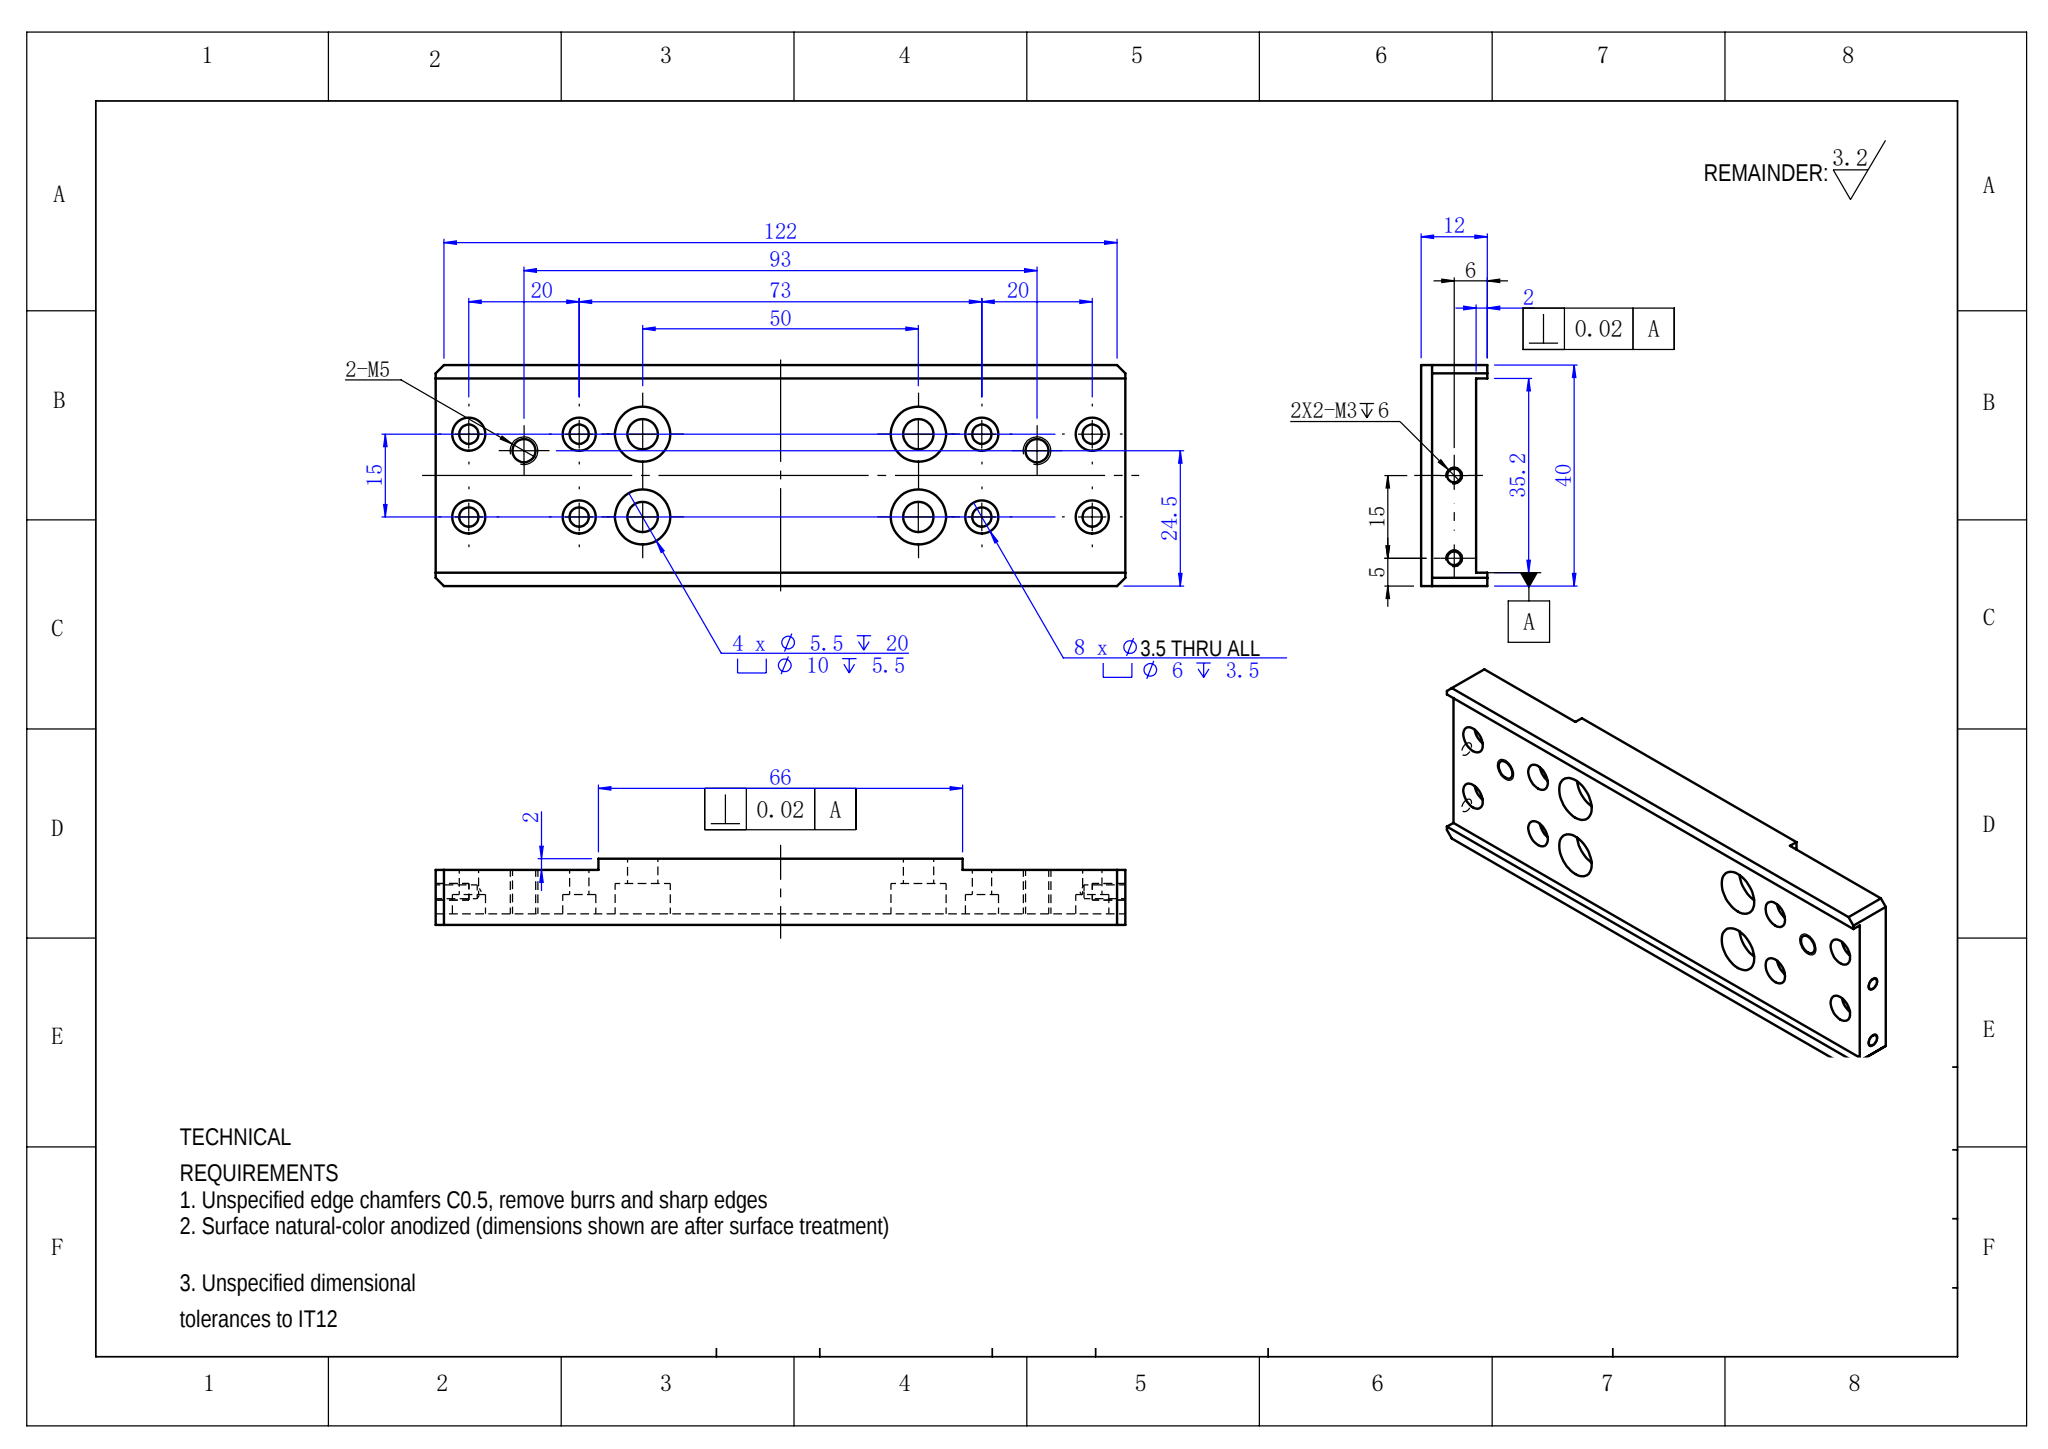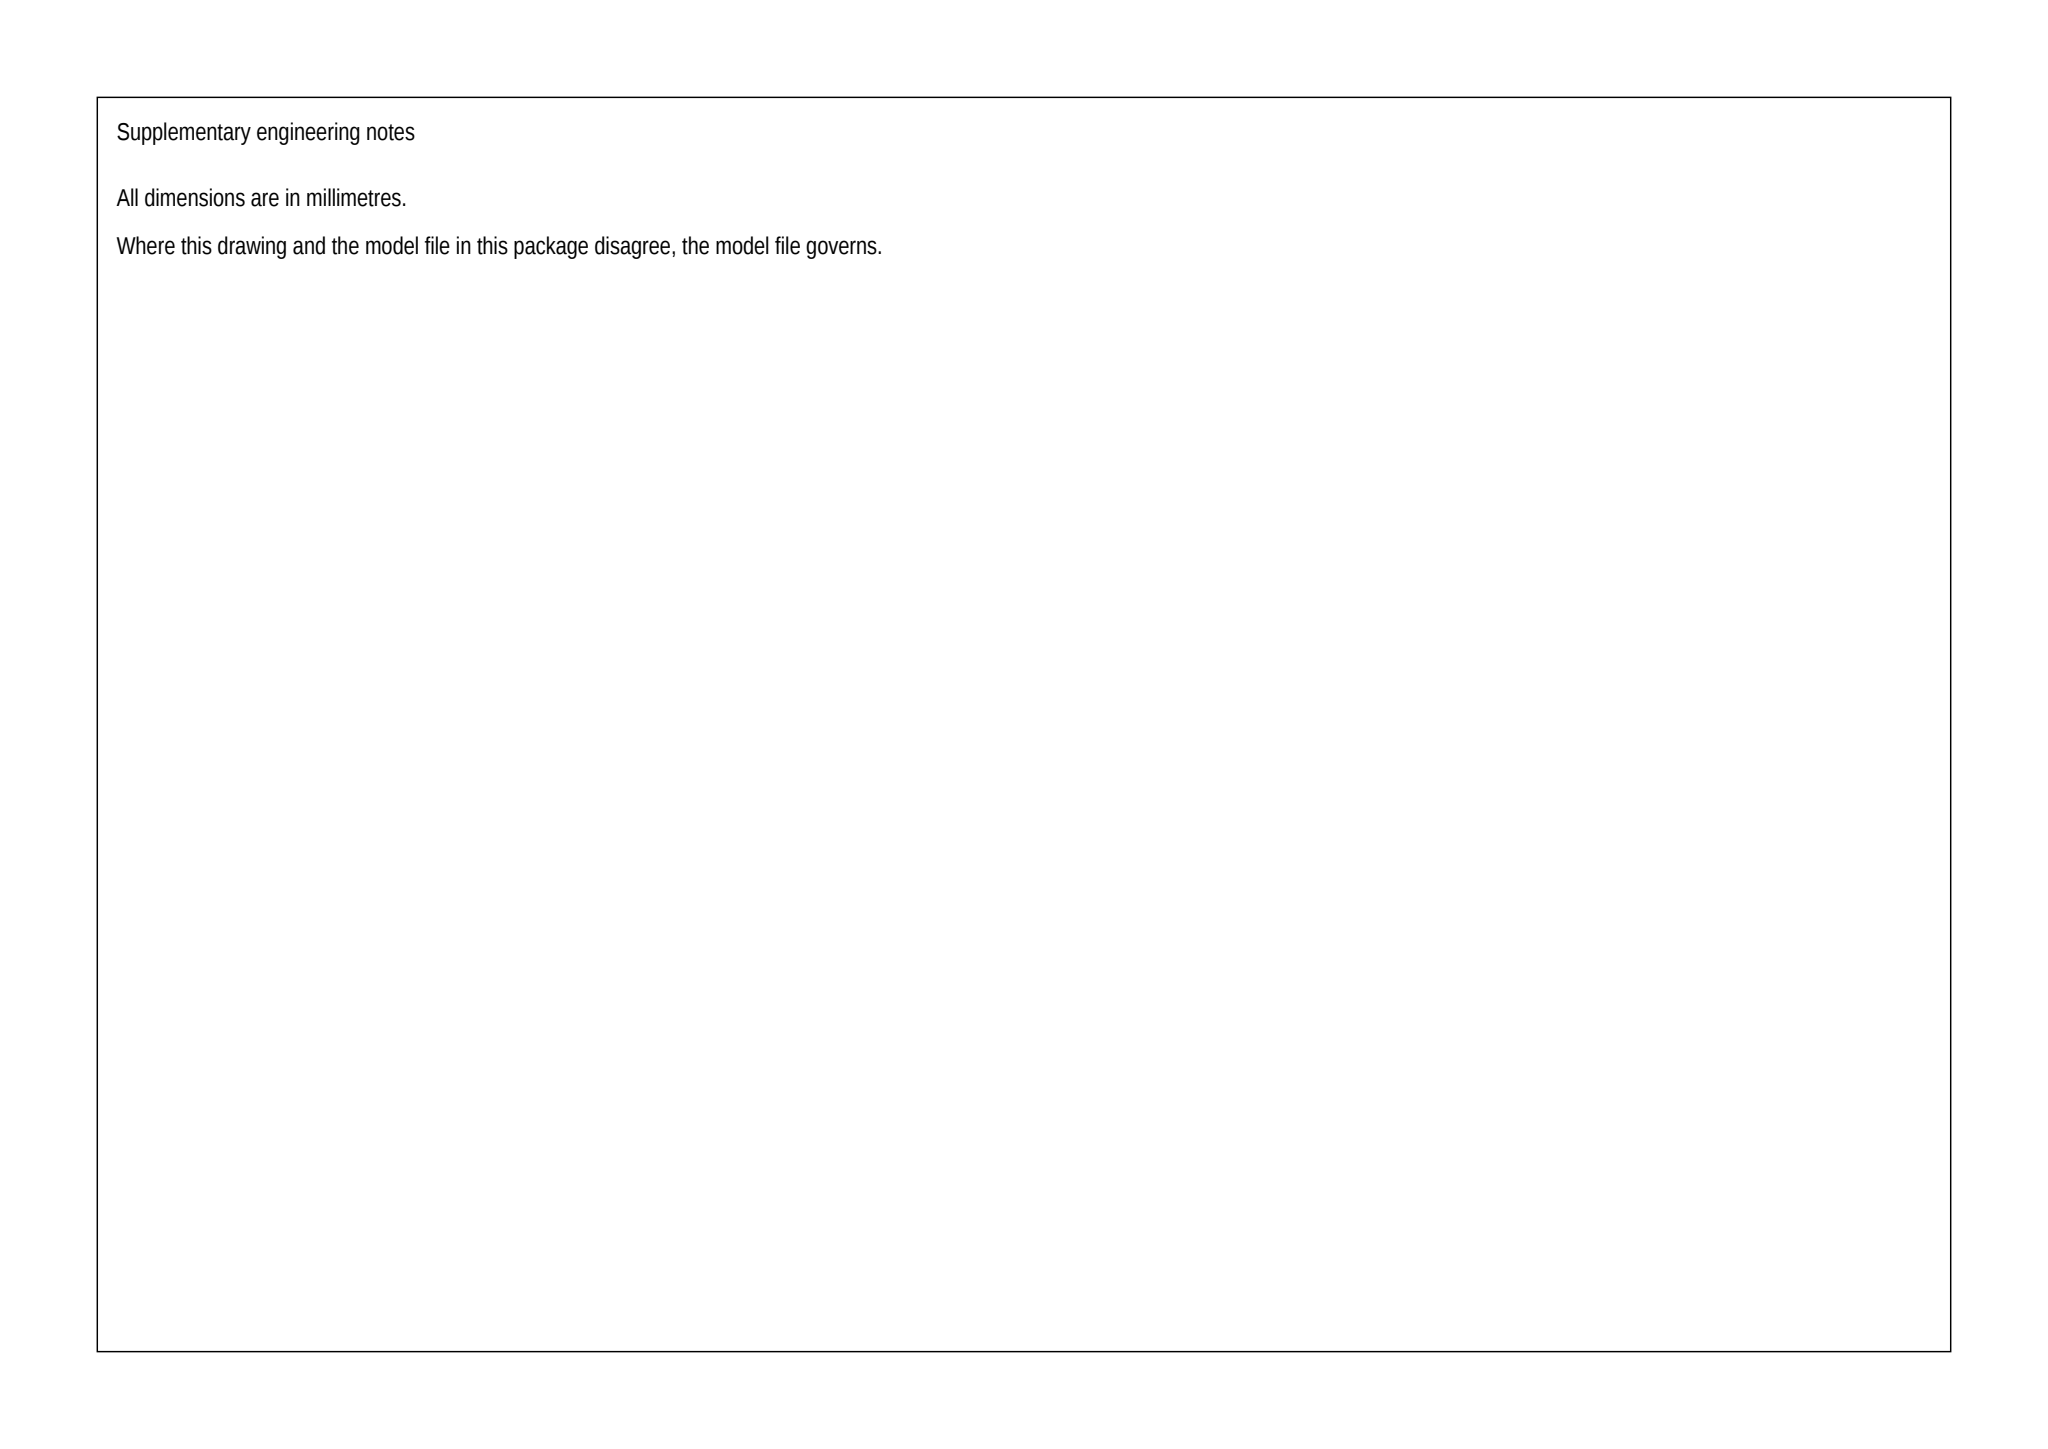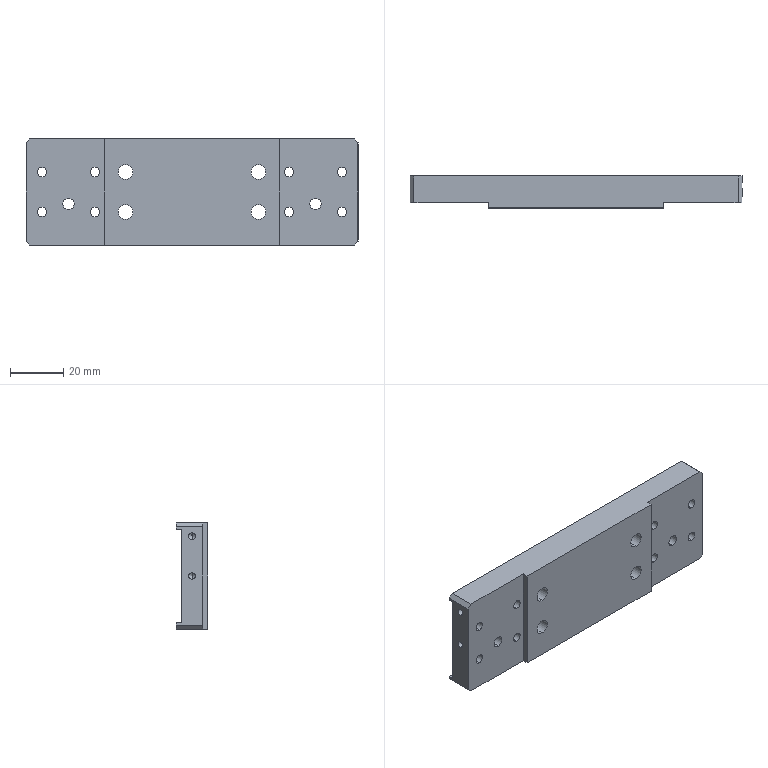Part | SolidWorks | mm | 1 solid | 98 faces | box 125 x 12 x 40 mm | volume 42768 mm3 | cylinder 60 | plane 30 | cone 8 | commonest cylinder face diameters 6 x16 3.5 x16 2.5 x8 10 x8 5.5 x8 4.2 x4
build123d program:
from build123d import *

# Parameters (mm, degrees)
SKETCH1_W                                         = 125
SKETCH1_H                                         = 40
BOSS_EXTRUDE1_DEPTH                               = 10
SKETCH2_W                                         = 29.5
SKETCH2_H                                         = 40
CUT_EXTRUDE1_DEPTH                                = 2
HOLE_SIZE_ACCORDING_TO_HEXAGON_SOCKET_D           = 5.5
HOLE_SIZE_ACCORDING_TO_HEXAGON_SOCKET_DEPTH       = 20
HOLE_SIZE_ACCORDING_TO_HEXAGON_SOCKET_CBORE_D     = 10
HOLE_SIZE_ACCORDING_TO_HEXAGON_SOCKET_CBORE_DEPTH = 5.5
HOLE_SIZE_ACCORDING_TO_HEXAGON_SOCKET_TIP         = 1.652
HOLE_SIZE_ACCORDING_TO_HEXAGON_SO_2_D             = 3.5
HOLE_SIZE_ACCORDING_TO_HEXAGON_SO_2_CBORE_D       = 6
HOLE_SIZE_ACCORDING_TO_HEXAGON_SO_2_CBORE_DEPTH   = 3.5
SKETCH8_W                                         = 125
SKETCH8_H                                         = 2.4
BOSS_EXTRUDE2_DEPTH                               = 2
M5_TAPPED_HOLE1_D                                 = 4.2
M3_TAPPED_HOLE1_AT_2_COUNT                        = 2
M3_TAPPED_HOLE1_AT_2_PITCH                        = 15
CHAMFER1_SIZE                                     = 1.5


with BuildPart() as part:
    # Sketch1 → Boss-Extrude1 (new body)
    with BuildSketch(Plane(origin=(0, 0, 0), x_dir=(1, 0, 0), z_dir=(0, 1, 0))):
        Rectangle(SKETCH1_W, SKETCH1_H)
    extrude(amount=BOSS_EXTRUDE1_DEPTH)

    # Sketch2 → Cut-Extrude1 (cut)
    with BuildSketch(Plane.XZ):
        with Locations((-47.75, 0)):
            Rectangle(SKETCH2_W, SKETCH2_H)
        with Locations((47.75, 0)):
            Rectangle(SKETCH2_W, SKETCH2_H)
    extrude(amount=-CUT_EXTRUDE1_DEPTH, mode=Mode.SUBTRACT)

    # Hole Size _ according to_ Hexagon Socket
    with Locations(Plane(origin=(0, 10, 0), x_dir=(1, 0, 0), z_dir=(0, 1, 0))):
        with Locations((-25, 7.5), (25, 7.5), (25, -7.5), (-25, -7.5)):
            CounterBoreHole(HOLE_SIZE_ACCORDING_TO_HEXAGON_SOCKET_D / 2, HOLE_SIZE_ACCORDING_TO_HEXAGON_SOCKET_CBORE_D / 2, HOLE_SIZE_ACCORDING_TO_HEXAGON_SOCKET_CBORE_DEPTH, depth=HOLE_SIZE_ACCORDING_TO_HEXAGON_SOCKET_DEPTH)
            with Locations((0, 0, -(HOLE_SIZE_ACCORDING_TO_HEXAGON_SOCKET_DEPTH + HOLE_SIZE_ACCORDING_TO_HEXAGON_SOCKET_TIP / 2))):  # 118° drill point
                Cone(0, HOLE_SIZE_ACCORDING_TO_HEXAGON_SOCKET_D / 2, HOLE_SIZE_ACCORDING_TO_HEXAGON_SOCKET_TIP, mode=Mode.SUBTRACT)

    # Hole Size _ according to_ Hexagon So 2 (through all)
    with Locations(Plane(origin=(0, 10, 0), x_dir=(1, 0, 0), z_dir=(0, 1, 0))):
        with Locations((-56.5, 7.5), (-36.5, 7.5), (-36.5, -7.5), (-56.5, -7.5), (56.5, -7.5), (36.5, -7.5), (36.5, 7.5), (56.5, 7.5)):
            CounterBoreHole(HOLE_SIZE_ACCORDING_TO_HEXAGON_SO_2_D / 2, HOLE_SIZE_ACCORDING_TO_HEXAGON_SO_2_CBORE_D / 2, HOLE_SIZE_ACCORDING_TO_HEXAGON_SO_2_CBORE_DEPTH)

    # Sketch8 → Boss-Extrude2 (add)
    with BuildSketch(Plane(origin=(0, 10, 0), x_dir=(1, 0, 0), z_dir=(0, 1, 0))):
        with Locations((0, 18.8)):
            Rectangle(SKETCH8_W, SKETCH8_H)
        with Locations((0, -18.8)):
            Rectangle(SKETCH8_W, SKETCH8_H)
    extrude(amount=BOSS_EXTRUDE2_DEPTH)

    # M5 Tapped Hole1 (through all)
    with Locations(Plane(origin=(0, 10, 0), x_dir=(1, 0, 0), z_dir=(0, 1, 0))):
        with Locations((-46.5, 4.5), (46.5, 4.5)):
            Hole(M5_TAPPED_HOLE1_D / 2)

    # Sketch12 → M3 Tapped Hole1 (revolve, cut)
    with BuildSketch(Plane(origin=(62.5, 6, 15), x_dir=(0, 0, -1), z_dir=(0, 1, 0))):
        Polygon((0, 0), (0, 8.251), (1.25, 7.5), (1.25, 0), align=None)
    m3_tapped_hole1 = revolve(axis=Axis((68.85, 6, 15), (-1, 0, 0)), mode=Mode.SUBTRACT)

    # M3 Tapped Hole1 at 2: M3 Tapped Hole1 ×2
    with Locations(*[(0, 0, -i * M3_TAPPED_HOLE1_AT_2_PITCH) for i in range(1, M3_TAPPED_HOLE1_AT_2_COUNT)]):
        add(m3_tapped_hole1, mode=Mode.SUBTRACT)

    # Mirror1: M3 Tapped Hole1 across plane
    add(m3_tapped_hole1.mirror(Plane(origin=(0, 0, 0), x_dir=(0, 0, 1), z_dir=(1, 0, 0))), mode=Mode.SUBTRACT)

    # Mirror1 copy 1 sketch → Mirror1 copy 1 (revolve, cut)
    with BuildSketch(Plane(origin=(-62.5, 6, 0), x_dir=(0, 0, -1), z_dir=(0, 1, 0))):
        Polygon((0, 0), (0, -8.251), (1.25, -7.5), (1.25, 0), align=None)
    revolve(axis=Axis((-68.85, 6, 0), (-1, 0, 0)), mode=Mode.SUBTRACT)

    # Chamfer1
    chamfer1_edges = [part.edges().sort_by_distance(p)[0] for p in [
        (62.5, 7, 20),
        (-62.5, 7, 20),
        (-62.5, 7, -20),
        (62.5, 7, -20),
    ]]
    chamfer(chamfer1_edges, length=CHAMFER1_SIZE)


solid = part.part